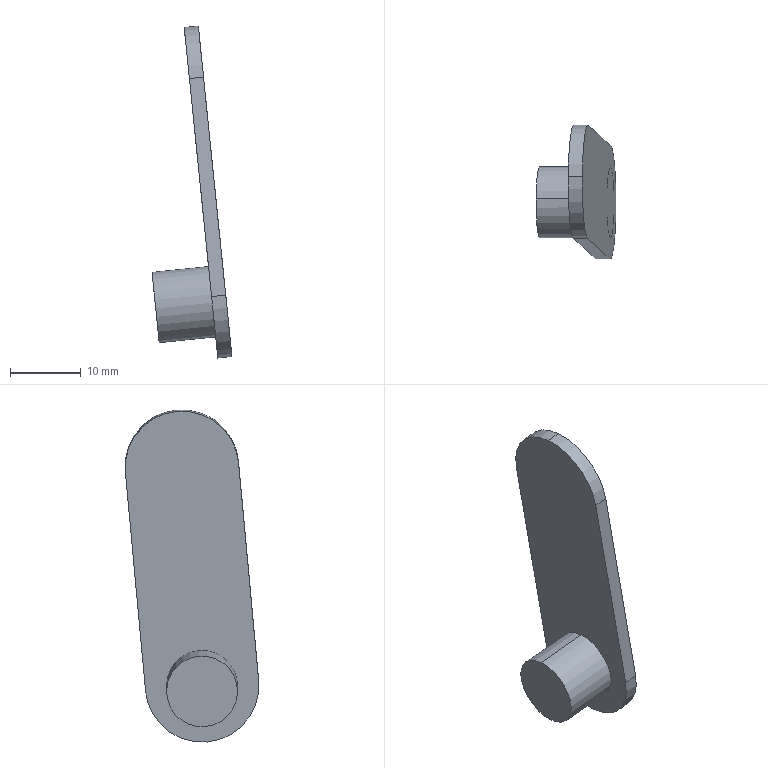Component | SolidWorks | Lock3-1 | 2 solids | 13 faces | box 11.26 x 18.83 x 46.83 mm | volume 2022 mm3 | cylinder 7 | plane 6 | commonest cylinder face diameters 10 x4 16 x3
STEP:
#1=COLOUR_RGB('',0.7922,0.8196,0.9333);
#2=FILL_AREA_STYLE_COLOUR('',#1);
#3=FILL_AREA_STYLE('',(#2));
#4=SURFACE_STYLE_FILL_AREA(#3);
#5=SURFACE_SIDE_STYLE('',(#4));
#6=SURFACE_STYLE_USAGE(.BOTH.,#5);
#7=PRESENTATION_STYLE_ASSIGNMENT((#6));
#8=CARTESIAN_POINT('',(-10.178,-2.503,23.905));
#9=VERTEX_POINT('',#8);
#10=CARTESIAN_POINT('',(-10.217,-2.467,24.295));
#11=VERTEX_POINT('',#10);
#12=CARTESIAN_POINT('',(-10.198,-2.485,24.1));
#13=DIRECTION('',(-0.9949,-0.,-0.1012));
#14=DIRECTION('',(0.1008,-0.09135,-0.9907));
#15=AXIS2_PLACEMENT_3D('',#12,#13,#14);
#16=CIRCLE('',#15,0.1969);
#17=EDGE_CURVE('',#9,#11,#16,.T.);
#18=ORIENTED_EDGE('',*,*,#17,.F.);
#19=CARTESIAN_POINT('',(-9.786,-2.503,23.945));
#20=VERTEX_POINT('',#19);
#21=CARTESIAN_POINT('',(-10.178,-2.503,23.905));
#22=DIRECTION('',(0.9949,0.,0.1012));
#23=VECTOR('',#22,39.37);
#24=LINE('',#21,#23);
#25=EDGE_CURVE('',#9,#20,#24,.T.);
#26=ORIENTED_EDGE('',*,*,#25,.T.);
#27=CARTESIAN_POINT('',(-9.826,-2.467,24.335));
#28=VERTEX_POINT('',#27);
#29=CARTESIAN_POINT('',(-9.806,-2.485,24.14));
#30=DIRECTION('',(-0.9949,-0.,-0.1012));
#31=DIRECTION('',(0.1008,-0.09135,-0.9907));
#32=AXIS2_PLACEMENT_3D('',#29,#30,#31);
#33=CIRCLE('',#32,0.1969);
#34=EDGE_CURVE('',#20,#28,#33,.T.);
#35=ORIENTED_EDGE('',*,*,#34,.T.);
#36=CARTESIAN_POINT('',(-10.217,-2.467,24.295));
#37=DIRECTION('',(0.9949,0.,0.1012));
#38=VECTOR('',#37,39.37);
#39=LINE('',#36,#38);
#40=EDGE_CURVE('',#11,#28,#39,.T.);
#41=ORIENTED_EDGE('',*,*,#40,.F.);
#42=EDGE_LOOP('',(#18,#26,#35,#41));
#43=FACE_OUTER_BOUND('',#42,.T.);
#44=CARTESIAN_POINT('',(-10.198,-2.485,24.1));
#45=DIRECTION('',(0.9949,0.,0.1012));
#46=DIRECTION('',(-0.1008,0.09135,0.9907));
#47=AXIS2_PLACEMENT_3D('',#44,#45,#46);
#48=CYLINDRICAL_SURFACE('',#47,0.1969);
#49=ADVANCED_FACE('',(#43),#48,.T.);
#50=ORIENTED_EDGE('',*,*,#25,.F.);
#51=CARTESIAN_POINT('',(-10.198,-2.485,24.1));
#52=DIRECTION('',(-0.9949,-0.,-0.1012));
#53=DIRECTION('',(0.1008,-0.09135,-0.9907));
#54=AXIS2_PLACEMENT_3D('',#51,#52,#53);
#55=CIRCLE('',#54,0.1969);
#56=EDGE_CURVE('',#11,#9,#55,.T.);
#57=ORIENTED_EDGE('',*,*,#56,.F.);
#58=ORIENTED_EDGE('',*,*,#40,.T.);
#59=CARTESIAN_POINT('',(-9.806,-2.485,24.14));
#60=DIRECTION('',(-0.9949,-0.,-0.1012));
#61=DIRECTION('',(0.1008,-0.09135,-0.9907));
#62=AXIS2_PLACEMENT_3D('',#59,#60,#61);
#63=CIRCLE('',#62,0.1969);
#64=EDGE_CURVE('',#28,#20,#63,.T.);
#65=ORIENTED_EDGE('',*,*,#64,.T.);
#66=EDGE_LOOP('',(#50,#57,#58,#65));
#67=FACE_OUTER_BOUND('',#66,.T.);
#68=CARTESIAN_POINT('',(-10.198,-2.485,24.1));
#69=DIRECTION('',(0.9949,0.,0.1012));
#70=DIRECTION('',(-0.1008,0.09135,0.9907));
#71=AXIS2_PLACEMENT_3D('',#68,#69,#70);
#72=CYLINDRICAL_SURFACE('',#71,0.1969);
#73=ADVANCED_FACE('',(#67),#72,.T.);
#74=ORIENTED_EDGE('',*,*,#56,.T.);
#75=ORIENTED_EDGE('',*,*,#17,.T.);
#76=EDGE_LOOP('',(#74,#75));
#77=FACE_OUTER_BOUND('',#76,.T.);
#78=CARTESIAN_POINT('',(-10.198,-2.485,24.1));
#79=DIRECTION('',(-0.9949,-0.,-0.1012));
#80=DIRECTION('',(0.1008,-0.09135,-0.9907));
#81=AXIS2_PLACEMENT_3D('',#78,#79,#80);
#82=PLANE('',#81);
#83=ADVANCED_FACE('',(#77),#82,.T.);
#84=ORIENTED_EDGE('',*,*,#64,.F.);
#85=ORIENTED_EDGE('',*,*,#34,.F.);
#86=EDGE_LOOP('',(#84,#85));
#87=FACE_OUTER_BOUND('',#86,.T.);
#88=CARTESIAN_POINT('',(-9.806,-2.485,24.14));
#89=DIRECTION('',(-0.9949,-0.,-0.1012));
#90=DIRECTION('',(0.1008,-0.09135,-0.9907));
#91=AXIS2_PLACEMENT_3D('',#88,#89,#90);
#92=PLANE('',#91);
#93=ADVANCED_FACE('',(#87),#92,.F.);
#94=CLOSED_SHELL('',(#49,#73,#83,#93));
#95=MANIFOLD_SOLID_BREP('',#94);
#96=STYLED_ITEM('',(#7),#95);
#97=(LENGTH_UNIT()NAMED_UNIT(*)SI_UNIT($,.METRE.));
#98=LENGTH_MEASURE_WITH_UNIT(LENGTH_MEASURE(0.0254),#97);
#99=DIMENSIONAL_EXPONENTS(1.,0.,0.,0.,0.,0.,0.);
#100=(CONVERSION_BASED_UNIT('',#98)LENGTH_UNIT()NAMED_UNIT(#99));
#101=UNCERTAINTY_MEASURE_WITH_UNIT(LENGTH_MEASURE(0.00001),#100,'','');
#102=(NAMED_UNIT(*)PLANE_ANGLE_UNIT()SI_UNIT($,.RADIAN.));
#103=(NAMED_UNIT(*)SI_UNIT($,.STERADIAN.)SOLID_ANGLE_UNIT());
#104=(GEOMETRIC_REPRESENTATION_CONTEXT(3)GLOBAL_UNCERTAINTY_ASSIGNED_CONTEXT((#101))GLOBAL_UNIT_ASSIGNED_CONTEXT((#100,#102,#103))REPRESENTATION_CONTEXT('',''));
#105=MECHANICAL_DESIGN_GEOMETRIC_PRESENTATION_REPRESENTATION('',(#96),#104);
#106=COLOUR_RGB('',0.7922,0.8196,0.9333);
#107=FILL_AREA_STYLE_COLOUR('',#106);
#108=FILL_AREA_STYLE('',(#107));
#109=SURFACE_STYLE_FILL_AREA(#108);
#110=SURFACE_SIDE_STYLE('',(#109));
#111=SURFACE_STYLE_USAGE(.BOTH.,#110);
#112=PRESENTATION_STYLE_ASSIGNMENT((#111));
#113=CARTESIAN_POINT('',(-9.864,-2.503,23.937));
#114=VERTEX_POINT('',#113);
#115=CARTESIAN_POINT('',(-9.904,-2.467,24.327));
#116=VERTEX_POINT('',#115);
#117=CARTESIAN_POINT('',(-9.884,-2.485,24.132));
#118=DIRECTION('',(0.9949,0.,0.1012));
#119=DIRECTION('',(-0.1008,0.09135,0.9907));
#120=AXIS2_PLACEMENT_3D('',#117,#118,#119);
#121=CIRCLE('',#120,0.1969);
#122=EDGE_CURVE('',#114,#116,#121,.T.);
#123=ORIENTED_EDGE('',*,*,#122,.F.);
#124=CARTESIAN_POINT('',(-9.786,-2.503,23.945));
#125=VERTEX_POINT('',#124);
#126=CARTESIAN_POINT('',(-9.864,-2.503,23.937));
#127=DIRECTION('',(0.9949,0.,0.1012));
#128=VECTOR('',#127,39.37);
#129=LINE('',#126,#128);
#130=EDGE_CURVE('',#114,#125,#129,.T.);
#131=ORIENTED_EDGE('',*,*,#130,.T.);
#132=CARTESIAN_POINT('',(-9.826,-2.467,24.335));
#133=VERTEX_POINT('',#132);
#134=CARTESIAN_POINT('',(-9.806,-2.485,24.14));
#135=DIRECTION('',(0.9949,0.,0.1012));
#136=DIRECTION('',(-0.1008,0.09135,0.9907));
#137=AXIS2_PLACEMENT_3D('',#134,#135,#136);
#138=CIRCLE('',#137,0.1969);
#139=EDGE_CURVE('',#125,#133,#138,.T.);
#140=ORIENTED_EDGE('',*,*,#139,.T.);
#141=CARTESIAN_POINT('',(-9.904,-2.467,24.327));
#142=DIRECTION('',(0.9949,0.,0.1012));
#143=VECTOR('',#142,39.37);
#144=LINE('',#141,#143);
#145=EDGE_CURVE('',#116,#133,#144,.T.);
#146=ORIENTED_EDGE('',*,*,#145,.F.);
#147=EDGE_LOOP('',(#123,#131,#140,#146));
#148=FACE_OUTER_BOUND('',#147,.T.);
#149=CARTESIAN_POINT('',(-9.884,-2.485,24.132));
#150=DIRECTION('',(0.9949,0.,0.1012));
#151=DIRECTION('',(-0.1008,0.09135,0.9907));
#152=AXIS2_PLACEMENT_3D('',#149,#150,#151);
#153=CYLINDRICAL_SURFACE('',#152,0.1969);
#154=ADVANCED_FACE('',(#148),#153,.F.);
#155=CARTESIAN_POINT('',(-10.004,-2.06,25.312));
#156=VERTEX_POINT('',#155);
#157=CARTESIAN_POINT('',(-10.039,-2.345,25.653));
#158=VERTEX_POINT('',#157);
#159=CARTESIAN_POINT('',(-10.007,-2.374,25.341));
#160=DIRECTION('',(0.9949,0.,0.1012));
#161=DIRECTION('',(-0.1008,0.09135,0.9907));
#162=AXIS2_PLACEMENT_3D('',#159,#160,#161);
#163=CIRCLE('',#162,0.315);
#164=EDGE_CURVE('',#156,#158,#163,.T.);
#165=ORIENTED_EDGE('',*,*,#164,.T.);
#166=CARTESIAN_POINT('',(-9.961,-2.345,25.661));
#167=VERTEX_POINT('',#166);
#168=CARTESIAN_POINT('',(-10.039,-2.345,25.653));
#169=DIRECTION('',(0.9949,0.,0.1012));
#170=VECTOR('',#169,39.37);
#171=LINE('',#168,#170);
#172=EDGE_CURVE('',#158,#167,#171,.T.);
#173=ORIENTED_EDGE('',*,*,#172,.T.);
#174=CARTESIAN_POINT('',(-9.926,-2.06,25.32));
#175=VERTEX_POINT('',#174);
#176=CARTESIAN_POINT('',(-9.929,-2.374,25.349));
#177=DIRECTION('',(0.9949,0.,0.1012));
#178=DIRECTION('',(-0.1008,0.09135,0.9907));
#179=AXIS2_PLACEMENT_3D('',#176,#177,#178);
#180=CIRCLE('',#179,0.315);
#181=EDGE_CURVE('',#175,#167,#180,.T.);
#182=ORIENTED_EDGE('',*,*,#181,.F.);
#183=CARTESIAN_POINT('',(-10.004,-2.06,25.312));
#184=DIRECTION('',(0.9949,0.,0.1012));
#185=VECTOR('',#184,39.37);
#186=LINE('',#183,#185);
#187=EDGE_CURVE('',#156,#175,#186,.T.);
#188=ORIENTED_EDGE('',*,*,#187,.F.);
#189=EDGE_LOOP('',(#165,#173,#182,#188));
#190=FACE_OUTER_BOUND('',#189,.T.);
#191=CARTESIAN_POINT('',(-10.007,-2.374,25.341));
#192=DIRECTION('',(0.9949,0.,0.1012));
#193=DIRECTION('',(-0.1008,0.09135,0.9907));
#194=AXIS2_PLACEMENT_3D('',#191,#192,#193);
#195=CYLINDRICAL_SURFACE('',#194,0.315);
#196=ADVANCED_FACE('',(#190),#195,.T.);
#197=ORIENTED_EDGE('',*,*,#172,.F.);
#198=CARTESIAN_POINT('',(-10.01,-2.688,25.369));
#199=VERTEX_POINT('',#198);
#200=CARTESIAN_POINT('',(-10.007,-2.374,25.341));
#201=DIRECTION('',(0.9949,0.,0.1012));
#202=DIRECTION('',(-0.1008,0.09135,0.9907));
#203=AXIS2_PLACEMENT_3D('',#200,#201,#202);
#204=CIRCLE('',#203,0.315);
#205=EDGE_CURVE('',#158,#199,#204,.T.);
#206=ORIENTED_EDGE('',*,*,#205,.T.);
#207=CARTESIAN_POINT('',(-9.932,-2.688,25.377));
#208=VERTEX_POINT('',#207);
#209=CARTESIAN_POINT('',(-10.01,-2.688,25.369));
#210=DIRECTION('',(0.9949,0.,0.1012));
#211=VECTOR('',#210,39.37);
#212=LINE('',#209,#211);
#213=EDGE_CURVE('',#199,#208,#212,.T.);
#214=ORIENTED_EDGE('',*,*,#213,.T.);
#215=CARTESIAN_POINT('',(-9.929,-2.374,25.349));
#216=DIRECTION('',(0.9949,0.,0.1012));
#217=DIRECTION('',(-0.1008,0.09135,0.9907));
#218=AXIS2_PLACEMENT_3D('',#215,#216,#217);
#219=CIRCLE('',#218,0.315);
#220=EDGE_CURVE('',#167,#208,#219,.T.);
#221=ORIENTED_EDGE('',*,*,#220,.F.);
#222=EDGE_LOOP('',(#197,#206,#214,#221));
#223=FACE_OUTER_BOUND('',#222,.T.);
#224=CARTESIAN_POINT('',(-10.007,-2.374,25.341));
#225=DIRECTION('',(0.9949,0.,0.1012));
#226=DIRECTION('',(-0.1008,0.09135,0.9907));
#227=AXIS2_PLACEMENT_3D('',#224,#225,#226);
#228=CYLINDRICAL_SURFACE('',#227,0.315);
#229=ADVANCED_FACE('',(#223),#228,.T.);
#230=CARTESIAN_POINT('',(-9.803,-2.172,24.111));
#231=VERTEX_POINT('',#230);
#232=CARTESIAN_POINT('',(-9.926,-2.06,25.32));
#233=DIRECTION('',(-0.1008,0.09135,0.9907));
#234=VECTOR('',#233,39.37);
#235=LINE('',#232,#234);
#236=EDGE_CURVE('',#231,#175,#235,.T.);
#237=ORIENTED_EDGE('',*,*,#236,.F.);
#238=CARTESIAN_POINT('',(-9.881,-2.172,24.103));
#239=VERTEX_POINT('',#238);
#240=CARTESIAN_POINT('',(-9.881,-2.172,24.103));
#241=DIRECTION('',(0.9949,0.,0.1012));
#242=VECTOR('',#241,39.37);
#243=LINE('',#240,#242);
#244=EDGE_CURVE('',#239,#231,#243,.T.);
#245=ORIENTED_EDGE('',*,*,#244,.F.);
#246=CARTESIAN_POINT('',(-10.004,-2.06,25.312));
#247=DIRECTION('',(-0.1008,0.09135,0.9907));
#248=VECTOR('',#247,39.37);
#249=LINE('',#246,#248);
#250=EDGE_CURVE('',#239,#156,#249,.T.);
#251=ORIENTED_EDGE('',*,*,#250,.T.);
#252=ORIENTED_EDGE('',*,*,#187,.T.);
#253=EDGE_LOOP('',(#237,#245,#251,#252));
#254=FACE_OUTER_BOUND('',#253,.T.);
#255=CARTESIAN_POINT('',(-10.004,-2.06,25.312));
#256=DIRECTION('',(0.009247,0.9958,-0.09089));
#257=DIRECTION('',(0.1008,-0.09135,-0.9907));
#258=AXIS2_PLACEMENT_3D('',#255,#256,#257);
#259=PLANE('',#258);
#260=ADVANCED_FACE('',(#254),#259,.T.);
#261=CARTESIAN_POINT('',(-9.809,-2.799,24.168));
#262=VERTEX_POINT('',#261);
#263=CARTESIAN_POINT('',(-9.806,-2.485,24.14));
#264=DIRECTION('',(0.9949,0.,0.1012));
#265=DIRECTION('',(-0.1008,0.09135,0.9907));
#266=AXIS2_PLACEMENT_3D('',#263,#264,#265);
#267=CIRCLE('',#266,0.315);
#268=EDGE_CURVE('',#262,#231,#267,.T.);
#269=ORIENTED_EDGE('',*,*,#268,.F.);
#270=CARTESIAN_POINT('',(-9.887,-2.799,24.16));
#271=VERTEX_POINT('',#270);
#272=CARTESIAN_POINT('',(-9.887,-2.799,24.16));
#273=DIRECTION('',(0.9949,0.,0.1012));
#274=VECTOR('',#273,39.37);
#275=LINE('',#272,#274);
#276=EDGE_CURVE('',#271,#262,#275,.T.);
#277=ORIENTED_EDGE('',*,*,#276,.F.);
#278=CARTESIAN_POINT('',(-9.884,-2.485,24.132));
#279=DIRECTION('',(0.9949,0.,0.1012));
#280=DIRECTION('',(-0.1008,0.09135,0.9907));
#281=AXIS2_PLACEMENT_3D('',#278,#279,#280);
#282=CIRCLE('',#281,0.315);
#283=EDGE_CURVE('',#271,#239,#282,.T.);
#284=ORIENTED_EDGE('',*,*,#283,.T.);
#285=ORIENTED_EDGE('',*,*,#244,.T.);
#286=EDGE_LOOP('',(#269,#277,#284,#285));
#287=FACE_OUTER_BOUND('',#286,.T.);
#288=CARTESIAN_POINT('',(-9.884,-2.485,24.132));
#289=DIRECTION('',(0.9949,0.,0.1012));
#290=DIRECTION('',(-0.1008,0.09135,0.9907));
#291=AXIS2_PLACEMENT_3D('',#288,#289,#290);
#292=CYLINDRICAL_SURFACE('',#291,0.315);
#293=ADVANCED_FACE('',(#287),#292,.T.);
#294=CARTESIAN_POINT('',(-9.932,-2.688,25.377));
#295=DIRECTION('',(0.1008,-0.09135,-0.9907));
#296=VECTOR('',#295,39.37);
#297=LINE('',#294,#296);
#298=EDGE_CURVE('',#208,#262,#297,.T.);
#299=ORIENTED_EDGE('',*,*,#298,.F.);
#300=ORIENTED_EDGE('',*,*,#213,.F.);
#301=CARTESIAN_POINT('',(-10.01,-2.688,25.369));
#302=DIRECTION('',(0.1008,-0.09135,-0.9907));
#303=VECTOR('',#302,39.37);
#304=LINE('',#301,#303);
#305=EDGE_CURVE('',#199,#271,#304,.T.);
#306=ORIENTED_EDGE('',*,*,#305,.T.);
#307=ORIENTED_EDGE('',*,*,#276,.T.);
#308=EDGE_LOOP('',(#299,#300,#306,#307));
#309=FACE_OUTER_BOUND('',#308,.T.);
#310=CARTESIAN_POINT('',(-10.01,-2.688,25.369));
#311=DIRECTION('',(-0.009247,-0.9958,0.09089));
#312=DIRECTION('',(-0.1008,0.09135,0.9907));
#313=AXIS2_PLACEMENT_3D('',#310,#311,#312);
#314=PLANE('',#313);
#315=ADVANCED_FACE('',(#309),#314,.T.);
#316=CARTESIAN_POINT('',(-9.884,-2.485,24.132));
#317=DIRECTION('',(0.9949,0.,0.1012));
#318=DIRECTION('',(-0.1008,0.09135,0.9907));
#319=AXIS2_PLACEMENT_3D('',#316,#317,#318);
#320=CIRCLE('',#319,0.1969);
#321=EDGE_CURVE('',#116,#114,#320,.T.);
#322=ORIENTED_EDGE('',*,*,#321,.T.);
#323=ORIENTED_EDGE('',*,*,#122,.T.);
#324=EDGE_LOOP('',(#322,#323));
#325=FACE_BOUND('',#324,.T.);
#326=ORIENTED_EDGE('',*,*,#164,.F.);
#327=ORIENTED_EDGE('',*,*,#250,.F.);
#328=ORIENTED_EDGE('',*,*,#283,.F.);
#329=ORIENTED_EDGE('',*,*,#305,.F.);
#330=ORIENTED_EDGE('',*,*,#205,.F.);
#331=EDGE_LOOP('',(#326,#327,#328,#329,#330));
#332=FACE_OUTER_BOUND('',#331,.T.);
#333=CARTESIAN_POINT('',(-10.007,-2.374,25.341));
#334=DIRECTION('',(0.9949,0.,0.1012));
#335=DIRECTION('',(-0.1008,0.09135,0.9907));
#336=AXIS2_PLACEMENT_3D('',#333,#334,#335);
#337=PLANE('',#336);
#338=ADVANCED_FACE('',(#325,#332),#337,.F.);
#339=CARTESIAN_POINT('',(-9.806,-2.485,24.14));
#340=DIRECTION('',(0.9949,0.,0.1012));
#341=DIRECTION('',(-0.1008,0.09135,0.9907));
#342=AXIS2_PLACEMENT_3D('',#339,#340,#341);
#343=CIRCLE('',#342,0.1969);
#344=EDGE_CURVE('',#133,#125,#343,.T.);
#345=ORIENTED_EDGE('',*,*,#344,.F.);
#346=ORIENTED_EDGE('',*,*,#139,.F.);
#347=EDGE_LOOP('',(#345,#346));
#348=FACE_BOUND('',#347,.T.);
#349=ORIENTED_EDGE('',*,*,#181,.T.);
#350=ORIENTED_EDGE('',*,*,#220,.T.);
#351=ORIENTED_EDGE('',*,*,#298,.T.);
#352=ORIENTED_EDGE('',*,*,#268,.T.);
#353=ORIENTED_EDGE('',*,*,#236,.T.);
#354=EDGE_LOOP('',(#349,#350,#351,#352,#353));
#355=FACE_OUTER_BOUND('',#354,.T.);
#356=CARTESIAN_POINT('',(-9.929,-2.374,25.349));
#357=DIRECTION('',(0.9949,0.,0.1012));
#358=DIRECTION('',(-0.1008,0.09135,0.9907));
#359=AXIS2_PLACEMENT_3D('',#356,#357,#358);
#360=PLANE('',#359);
#361=ADVANCED_FACE('',(#348,#355),#360,.T.);
#362=ORIENTED_EDGE('',*,*,#130,.F.);
#363=ORIENTED_EDGE('',*,*,#321,.F.);
#364=ORIENTED_EDGE('',*,*,#145,.T.);
#365=ORIENTED_EDGE('',*,*,#344,.T.);
#366=EDGE_LOOP('',(#362,#363,#364,#365));
#367=FACE_OUTER_BOUND('',#366,.T.);
#368=CARTESIAN_POINT('',(-9.884,-2.485,24.132));
#369=DIRECTION('',(0.9949,0.,0.1012));
#370=DIRECTION('',(-0.1008,0.09135,0.9907));
#371=AXIS2_PLACEMENT_3D('',#368,#369,#370);
#372=CYLINDRICAL_SURFACE('',#371,0.1969);
#373=ADVANCED_FACE('',(#367),#372,.F.);
#374=CLOSED_SHELL('',(#154,#196,#229,#260,#293,#315,#338,#361,#373));
#375=MANIFOLD_SOLID_BREP('',#374);
#376=STYLED_ITEM('',(#112),#375);
#377=(LENGTH_UNIT()NAMED_UNIT(*)SI_UNIT($,.METRE.));
#378=LENGTH_MEASURE_WITH_UNIT(LENGTH_MEASURE(0.0254),#377);
#379=DIMENSIONAL_EXPONENTS(1.,0.,0.,0.,0.,0.,0.);
#380=(CONVERSION_BASED_UNIT('',#378)LENGTH_UNIT()NAMED_UNIT(#379));
#381=UNCERTAINTY_MEASURE_WITH_UNIT(LENGTH_MEASURE(0.00001),#380,'','');
#382=(NAMED_UNIT(*)PLANE_ANGLE_UNIT()SI_UNIT($,.RADIAN.));
#383=(NAMED_UNIT(*)SI_UNIT($,.STERADIAN.)SOLID_ANGLE_UNIT());
#384=(GEOMETRIC_REPRESENTATION_CONTEXT(3)GLOBAL_UNCERTAINTY_ASSIGNED_CONTEXT((#381))GLOBAL_UNIT_ASSIGNED_CONTEXT((#380,#382,#383))REPRESENTATION_CONTEXT('',''));
#385=MECHANICAL_DESIGN_GEOMETRIC_PRESENTATION_REPRESENTATION('',(#376),#384);
#386=PRESENTATION_LAYER_ASSIGNMENT('','',(#376));
#387=PRESENTATION_LAYER_ASSIGNMENT('','',(#96));
#388=CARTESIAN_POINT('',(0.,0.,0.));
#389=DIRECTION('',(0.,0.,1.));
#390=DIRECTION('',(1.,0.,0.));
#391=AXIS2_PLACEMENT_3D('',#388,#389,#390);
#392=(LENGTH_UNIT()NAMED_UNIT(*)SI_UNIT($,.METRE.));
#393=LENGTH_MEASURE_WITH_UNIT(LENGTH_MEASURE(0.0254),#392);
#394=DIMENSIONAL_EXPONENTS(1.,0.,0.,0.,0.,0.,0.);
#395=(CONVERSION_BASED_UNIT('',#393)LENGTH_UNIT()NAMED_UNIT(#394));
#396=UNCERTAINTY_MEASURE_WITH_UNIT(LENGTH_MEASURE(0.00001),#395,'','');
#397=(NAMED_UNIT(*)PLANE_ANGLE_UNIT()SI_UNIT($,.RADIAN.));
#398=(NAMED_UNIT(*)SI_UNIT($,.STERADIAN.)SOLID_ANGLE_UNIT());
#399=(GEOMETRIC_REPRESENTATION_CONTEXT(3)GLOBAL_UNCERTAINTY_ASSIGNED_CONTEXT((#396))GLOBAL_UNIT_ASSIGNED_CONTEXT((#395,#397,#398))REPRESENTATION_CONTEXT('',''));
#400=ADVANCED_BREP_SHAPE_REPRESENTATION('',(#375,#95,#391),#399);